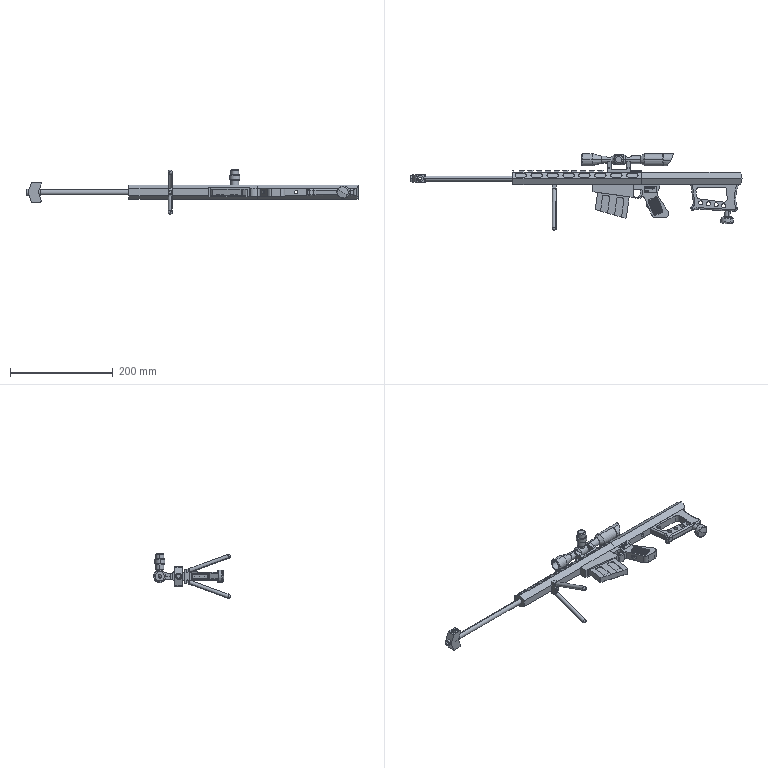Assembly | SolidWorks | mm | 18 component files | 18 solids | 1601 faces | box 645 x 149.11 x 86.63 mm | volume 407646 mm3 | plane 722 | cylinder 529 | spline 237 | cone 82 | torus 25 | sphere 6 | commonest cylinder face diameters 2 x243 10 x44 8 x42 6 x40 12 x33 6.5 x18 16 x14 5 x14
Bill of materials:
AdjustmentKnob | 1 |  | Stepped solid cylindrical pin with a rounded-edge top section, a wider chamfered collar, a main cylindrical body, and a reduced-diameter end spigot with a narrow groove and chamfered tip.
Barrel | 1 |  | Long slender hollow tube or rod. One end has a slightly larger-diameter section with a cross hole through it. The other end steps down to a smaller diameter with a groove and an open bore.
Bipod | 2 |  | Slender cylindrical pin with a hemispherical rounded end. The opposite end has a short reduced-diameter stub with a groove.
Bracket | 1 |  | U-shaped (channel) block: a base bar with two upright side arms. The base has a central through-hole. The arms flare outward in plan and have concave curved cutouts and notches at their ends.
Bullet | 3 |  | Elongated revolved body with a pointed ogive-shaped tip, stepped neck and shoulder, a long cylindrical body, a groove near the base, and a flat-ended rim. The overall profile resembles a cartridge shape.
ConnectingBlock | 1 |  | Rectangular block with one side angled into a shallow V-shaped (chevron) profile, and three round through-holes spaced along its length.
Eyepiece | 1 |  | Thin-walled cylindrical sleeve or ring with one end cut square and chamfered, and the other end cut at a steep curved/oblique angle.
Foot | 1 |  | Knob or stepped pin with a large rounded-edge disc head, a short collar, a cylindrical shank, and a smaller end spigot with a groove and chamfered tip.
Grip | 1 |  | Flat plate-like body with a pistol-shaped outline: a long rectangular upper section with a recessed open slot, a rounded through-opening in the middle, and an angled grip section with a dimpled texture pattern and raised text on one face.
LowerReceiver | 1 |  | Long hexagonal bar with a reduced cylindrical spigot at one end. Several small transverse holes run along it, including one through the spigot. The opposite end is rounded/chamfered.
Magazine | 1 |  | Flat rectangular slab with rounded corners, a slightly skewed outline, and stepped notches along one edge. Two shallow L-shaped grooves with rounded bends run across the top face.
MuzzleBrake | 1 |  | Block bent into a chevron (V) profile with rounded edges. One end face has a counterbored hole, and a side face has a cylindrical cross-hole with a large concave recess or spot-face around it.
Scope | 1 |  | Elongated turned (axisymmetric) tubular part. It has a larger-diameter cylindrical section at each end, joined by conical tapers to a narrower central shank. The middle of the shank has a short raised collar with chamfered edges. The shank has small cross holes on both sides of the collar and a larger cross hole through the collar. One end has a reduced-diameter stepped spigot with a small groove or step and an open axial bore.
Stock | 1 |  | Flat, roughly rectangular plate or bracket with rounded edges. It has a large rounded-rectangle through-window and a row of four round through-holes along one long side. The long sides have concave (inward-curving) edges, and one corner has a small projecting tab or lip. There is a small hole on the floor or wall inside the window area and a round hole in one end face, which appears to be counterbored or countersunk.
UpperReceiver | 1 |  | Long straight prismatic bar with a mainly hexagonal cross-section and a rectangular key-like protrusion along one flat. A large rounded, roughly circular bore runs through it lengthwise. One face has a regular row of elongated, slot-like shallow recesses, and there is a raised row of small rectangular teeth or notches along one edge. Two small round cross holes go through a side face.
Mates:
1. concentric | Grip-1 face at (49.182, 12.483, 1009) dir (0, 1, 0) r 4 | LowerReceiver-1 face at (49.182, 46.483, 1009) dir (0, 1, 0) r 3.25
2. coincident | Grip-1 face at (-65.818, 22.483, 1017) dir (0, 1, 0) | LowerReceiver-1 face at (29.182, 22.483, 1002.072) dir (0, -1, 0)
3. parallel | Grip-1 edge at (13.21, 22.483, 1017) dir (1, 0, 0) | LowerReceiver-1 edge at (29.182, 22.483, 1015.928) dir (1, 0, 0)
4. concentric | LowerReceiver-1 face at (201.182, 46.483, 1009) dir (0, 1, 0) r 3.25 | Stock-1 face at (201.182, 22.483, 1009) dir (0, 1, 0) r 2.5
5. coincident | LowerReceiver-1 face at (29.182, 22.483, 1002.072) dir (0, -1, 0) | Stock-1 face at (217.782, 22.483, 1016) dir (0, 1, 0)
6. parallel | LowerReceiver-1 edge at (29.182, 22.483, 1015.928) dir (1, 0, 0) | Stock-1 edge at (214.485, 22.483, 1016) dir (-1, 0, 0)
7. concentric | Stock-1 face at (196.272, -28.274, 1009) dir (-0.05643, -0.9984, 0) r 4.5 | Foot-1 face at (194.855, -53.332, 1009) dir (-0.05643, -0.9984, 0) r 4
8. lock | Stock-1 reference at (0, 0, 0) dir (1, 0, 0) | Foot-1 reference at (0, 0, 0) dir (1, 0, 0)
9. concentric | LowerReceiver-1 face at (9.182, 34.483, 1009) dir (1, 0, 0) r 9 | UpperReceiver-1 face at (8.182, 34.483, 1009) dir (1, 0, 0) r 9
10. coincident | LowerReceiver-1 face at (29.182, 34.483, 1009) dir (-1, 0, 0) | UpperReceiver-1 face at (29.182, 34.483, 1009) dir (1, 0, 0)
11. coincident | LowerReceiver-1 edge at (29.182, 46.483, 1015.928) dir (1, 0, 0) | UpperReceiver-1 edge at (29.182, 46.483, 1015.928) dir (-1, 0, 0)
12. concentric | UpperReceiver-1 face at (-15.318, 31.483, 1009) dir (0, 1, 0) r 3 | Bracket-1 face at (-15.318, 46.483, 1009) dir (0, 1, 0) r 3.5
13. coincident | UpperReceiver-1 face at (29.182, 46.483, 1002.072) dir (0, 1, 0) | Bracket-1 face at (-15.318, 46.483, 1009) dir (0, -1, 0)
14. parallel | UpperReceiver-1 edge at (29.182, 46.483, 1015.928) dir (-1, 0, 0) | Bracket-1 edge at (6.182, 46.483, 1015) dir (-1, 0, 0)
15. concentric | Bracket-1 face at (-34.068, 62.483, 1009) dir (0, 1, 0) r 2.5 | Scope-1 face at (-34.068, 53.983, 1009) dir (0, 1, 0) r 3.25
16. tangent | Bracket-1 face at (-30.318, 70.483, 1009) dir (-1, 0, 0) r 7.5 | Scope-1 face at (248.891, 70.983, 1008.111) dir (1, 0, -0.003141) r 7
17. lock | Bracket-1 reference at (0, 0, 0) dir (1, 0, 0) | Scope-1 reference at (0, 0, 0) dir (1, 0, 0)
18. concentric | UpperReceiver-1 face at (-140.818, 37.483, 1009) dir (0, -1, 0) r 3.5 | ConnectingBlock-1 face at (-140.818, 25.483, 1009) dir (0, -1, 0) r 3
19. coincident | UpperReceiver-1 face at (29.182, 22.483, 1015.928) dir (0, -1, 0) | ConnectingBlock-1 face at (-144.818, 22.483, 1023) dir (0, 1, 0)
20. perpendicular | UpperReceiver-1 edge at (29.182, 22.483, 1015.928) dir (-1, 0, 0) | ConnectingBlock-1 edge at (-144.818, 22.483, 1023) dir (0, 0, -1)
21. concentric | ConnectingBlock-1 face at (-140.818, 27.142, 1015.265) dir (0, -0.9397, 0.342) r 3 | Bipod-1 face at (-140.818, 19.624, 1018.001) dir (0, 0.9397, -0.342) r 3
22. coincident | ConnectingBlock-1 face at (-144.818, 16.123, 1023) dir (0, -0.9397, 0.342) | Bipod-1 face at (-142.875, 15.672, 1021.763) dir (0, -0.9397, 0.342)
23. concentric | ConnectingBlock-1 face at (-140.818, 27.142, 1002.735) dir (0, -0.9397, -0.342) r 3 | Bipod-2 face at (-140.818, 19.624, 999.999) dir (0, 0.9397, 0.342) r 3
24. coincident | ConnectingBlock-1 face at (-144.818, 12.483, 1005) dir (0, -0.9397, -0.342) | Bipod-2 face at (-138.423, 15.544, 996.591) dir (0, -0.9397, -0.342)
25. concentric | UpperReceiver-1 face at (-195.818, 34.483, 1009) dir (-1, 0, 0) r 4 | Barrel-1 face at (-420.818, 34.483, 1009) dir (-1, 0, 0) r 4
26. coincident | UpperReceiver-1 face at (-220.818, 34.483, 1009) dir (-1, 0, 0) | Barrel-1 face at (-220.818, 39.483, 1009) dir (1, 0, 0)
27. concentric | Barrel-1 face at (-420.818, 34.483, 1009) dir (-1, 0, 0) r 6 | MuzzleBrake-1 face at (-385.008, 34.483, 1009) dir (-1, 0, 0) r 6
28. concentric | Barrel-1 face at (-400.818, 34.483, 1028) dir (0, 0, -1) r 3 | MuzzleBrake-1 face at (-400.818, 34.483, 1028) dir (0, 0, 1) r 3
29. lock | Barrel-1 reference at (0, 0, 0) dir (1, 0, 0) | MuzzleBrake-1 reference at (0, 0, 0) dir (1, 0, 0)
30. lock | UpperReceiver-1 reference at (0, 0, 0) dir (1, 0, 0) | MuzzleBrake-1 reference at (0, 0, 0) dir (1, 0, 0)
31. concentric | Scope-1 face at (248.891, 70.983, 1008.111) dir (1, 0, -0.003141) r 10 | Eyepiece-1 face at (90.932, 70.983, 1008.607) dir (-1, 0, 0.003141) r 10
32. coincident | Scope-1 face at (69.959, 70.983, 1017.173) dir (1, 0, -0.003141) | Eyepiece-1 edge at (69.932, 70.983, 1008.673) dir (-1, 0, 0.003141) r 11
33. lock | Scope-1 reference at (0, 0, 0) dir (1, 0, 0) | Eyepiece-1 reference at (0, 0, 0) dir (1, 0, 0)
34. concentric | Scope-1 face at (-15.386, 70.983, 1018.941) dir (0.003141, 0, 1) r 6 | AdjustmentKnob-1 face at (-15.28, 70.983, 1052.851) dir (0.003141, 0, 1) r 6
35. lock | Scope-1 reference at (0, 0, 0) dir (1, 0, 0) | AdjustmentKnob-1 reference at (0, 0, 0) dir (1, 0, 0)
36. width | Magazine-1 face at (-61.023, -26.033, 1015) dir (0, 0, 1) | Magazine-1 face at (-61.023, -26.033, 1003) dir (0, 0, -1) | Grip-1 face at (249.605, 1778.063, 1000) dir (0, 0, -1) | Grip-1 face at (249.605, 1778.063, 1018) dir (0, 0, 1)
37. coincident | Magazine-1 face at (-1.05, -30.422, 1013) dir (-0.9903, 0.1392, 0) | Bullet-1 face at (-0.1726, -24.177, 1009.12) dir (0.9903, -0.1392, 0)
38. lock | Magazine-1 reference at (0, 0, 0) dir (1, 0, 0) | Bullet-1 reference at (0, 0, 0) dir (1, 0, 0)
39. coincident | Magazine-1 face at (-1.05, -30.422, 1013) dir (-0.9903, 0.1392, 0) | Bullet-3 face at (1.182, -14.538, 1009.095) dir (0.9903, -0.1392, 0)
40. lock | Magazine-1 reference at (0, 0, 0) dir (1, 0, 0) | Bullet-3 reference at (0, 0, 0) dir (1, 0, 0)
41. coincident | Magazine-1 face at (-1.05, -30.422, 1013) dir (-0.9903, 0.1392, 0) | Bullet-2 face at (2.615, -4.34, 1008.869) dir (0.9903, -0.1392, 0)
42. lock | Magazine-1 reference at (0, 0, 0) dir (1, 0, 0) | Bullet-2 reference at (0, 0, 0) dir (1, 0, 0)
43. coincident | Grip-1 face at (-66.844, 15.178, 1009) dir (-0.1392, -0.9903, 0) | Magazine-1 face at (-55.456, 13.578, 1015) dir (0.1392, 0.9903, 0)
44. lock | ConnectingBlock-1 reference at (0, 0, 0) dir (1, 0, 0) | Bipod-1 reference at (0, 0, 0) dir (1, 0, 0)
45. lock | ConnectingBlock-1 reference at (0, 0, 0) dir (1, 0, 0) | Bipod-2 reference at (0, 0, 0) dir (1, 0, 0)
46. width | Magazine-1 face at (-61.023, -26.033, 1015) dir (-0.9903, 0.1392, 0) | Magazine-1 face at (5.94, 4.949, 1015) dir (0.9903, -0.1392, 0) | Grip-1 face at (-58.922, 14.065, 1015) dir (0.9903, -0.1392, 0) | Grip-1 face at (9.406, 4.462, 1015) dir (-0.9903, 0.1392, 0)